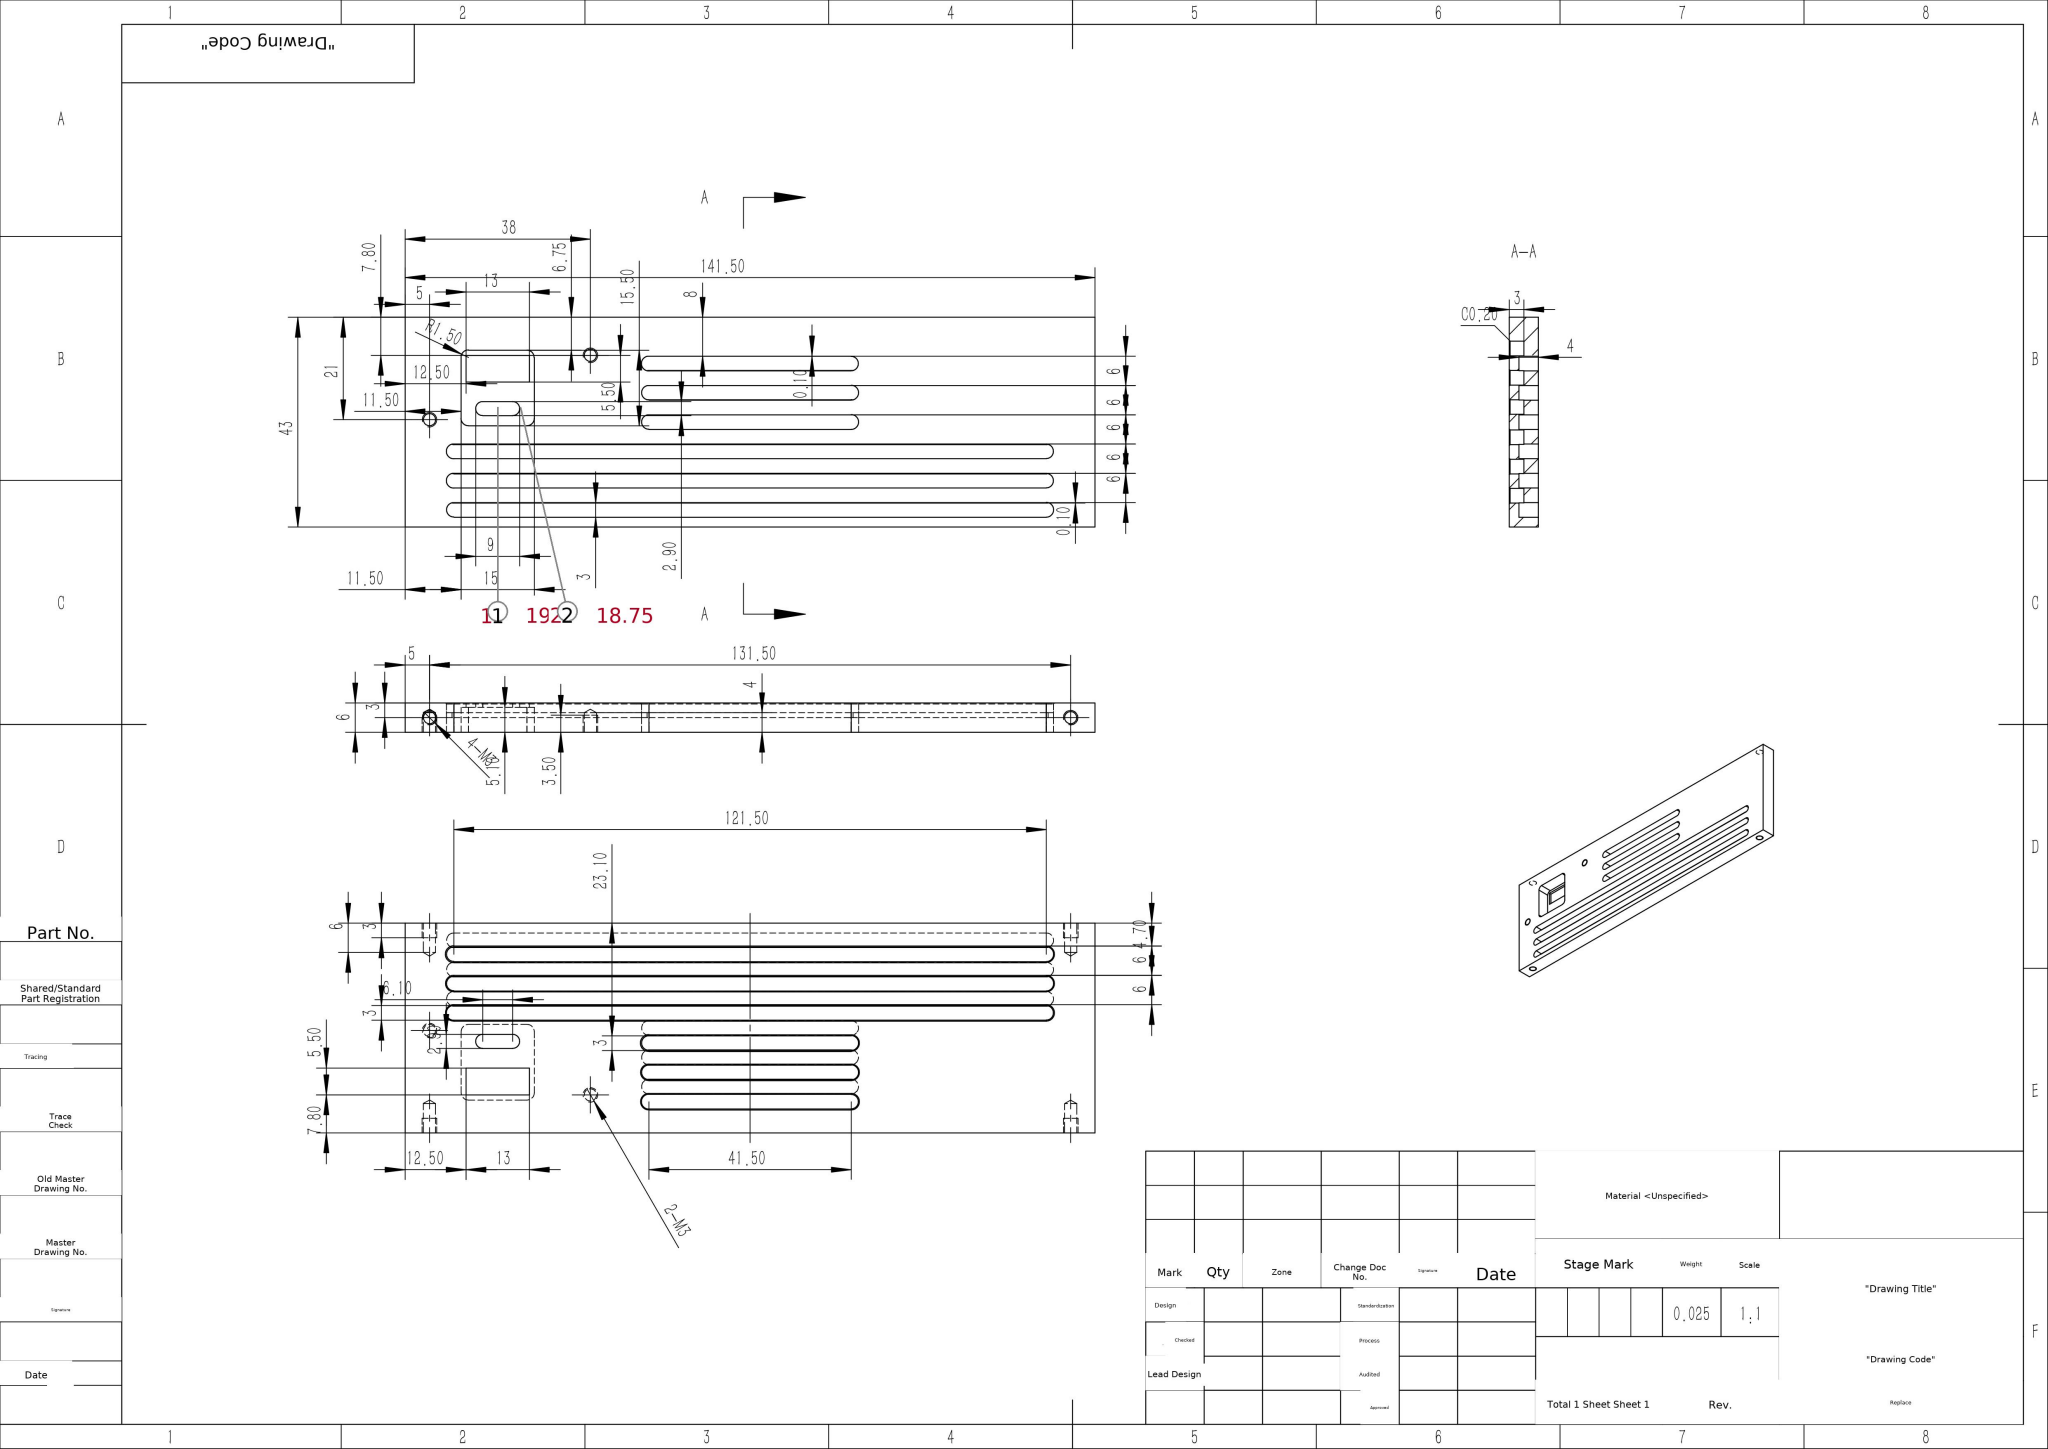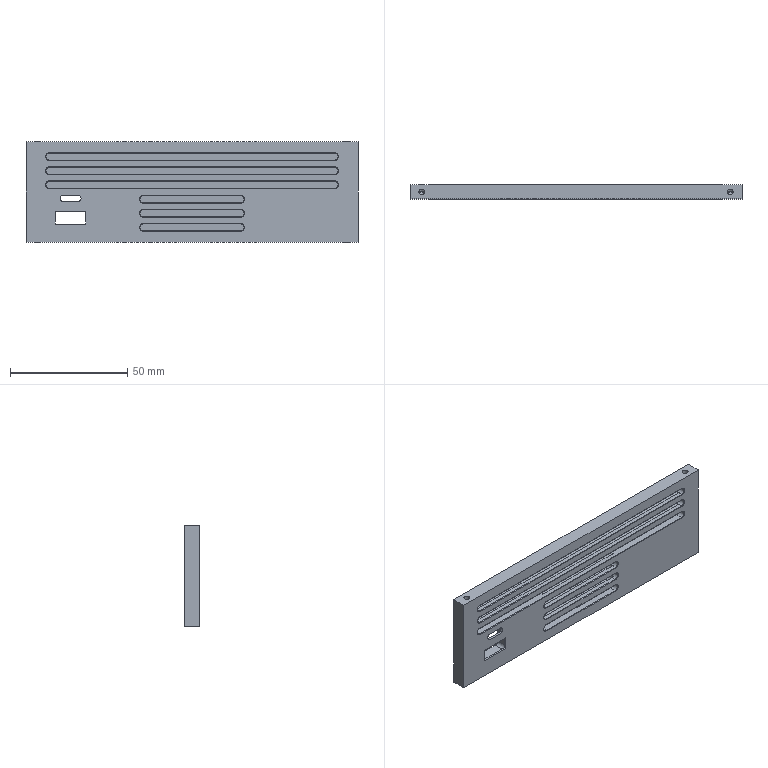Part | SolidWorks | mm | 1 solid | 131 faces | box 141.5 x 6 x 43 mm | volume 24539 mm3 | plane 65 | cylinder 42 | cone 24 | commonest cylinder face diameters 3 x28 2.5 x12 2.9 x2
build123d program:
from build123d import *

# Parameters (mm, degrees)
SKETCH1_W             = 141.5
SKETCH1_H             = 43
BOSS_EXTRUDE1_DEPTH   = 6
CUT_EXTRUDE1_DEPTH    = 4
LPATTERN1_COUNT       = 3
LPATTERN1_PITCH       = 6
CUT_EXTRUDE4_DEPTH    = 3
LPATTERN2_COUNT       = 3
LPATTERN2_PITCH       = 6
CUT_EXTRUDE5_DEPTH    = 4
LPATTERN3_COUNT       = 3
LPATTERN3_PITCH       = 6
CUT_EXTRUDE6_DEPTH    = 3
LPATTERN4_COUNT       = 3
LPATTERN4_PITCH       = 6
SKETCH13_W            = 15
SKETCH13_H            = 15.5
CUT_EXTRUDE7_DEPTH    = 5.1
FILLET1_R             = 1.5
CHAMFER2_SIZE         = 0.2
SKETCH15_W            = 13
SKETCH15_H            = 5.5
CUT_EXTRUDE8_DEPTH    = 5.1
CUT_EXTRUDE9_DEPTH    = 5.1
M3_TAPPED_HOLE3_D     = 2.5
M3_TAPPED_HOLE3_DEPTH = 4
M3_TAPPED_HOLE3_TIP   = 0.7511
M3_TAPPED_HOLE4_D     = 2.5
M3_TAPPED_HOLE4_DEPTH = 4
M3_TAPPED_HOLE4_TIP   = 0.7511


with BuildPart() as part:
    # Sketch1 → Boss-Extrude1 (new body)
    with BuildSketch(Plane(origin=(0, 0, 0), x_dir=(1, 0, 0), z_dir=(0, 1, 0))):
        Rectangle(SKETCH1_W, SKETCH1_H)
    extrude(amount=BOSS_EXTRUDE1_DEPTH)

    # Sketch5 → M3 Tapped Hole1 (revolve, cut)
    with BuildSketch(Plane(origin=(-65.75, 3, -21.5), x_dir=(0, 1, 0), z_dir=(1, 0, 0))):
        Polygon((0, 0), (0, 6.751), (1.25, 6), (1.25, 0), align=None)
    m3_tapped_hole1 = revolve(axis=Axis((-65.75, 3, -27.85), (0, 0, 1)), mode=Mode.SUBTRACT)

    # Sketch7 → M3 Tapped Hole2 (revolve, cut)
    with BuildSketch(Plane(origin=(-65.75, 3, 21.5), x_dir=(0, -1, 0), z_dir=(1, 0, 0))):
        Polygon((0, 0), (0, 6.751), (1.25, 6), (1.25, 0), align=None)
    m3_tapped_hole2 = revolve(axis=Axis((-65.75, 3, 27.85), (0, 0, -1)), mode=Mode.SUBTRACT)

    # Sketch9 → Cut-Extrude1 (cut)
    with BuildSketch(Plane(origin=(0, 6, 0), x_dir=(1, 0, 0), z_dir=(0, 1, 0))):
        with BuildLine():
            Line((60.75, -19.5), (-60.75, -19.5))
            ThreePointArc((-60.75, -19.5), (-62.25, -18), (-60.75, -16.5))
            Line((-60.75, -16.5), (60.75, -16.5))
            ThreePointArc((60.75, -16.5), (62.25, -18), (60.75, -19.5))
        make_face()
    cut_extrude1 = extrude(amount=-CUT_EXTRUDE1_DEPTH, mode=Mode.SUBTRACT)

    # LPattern1: Cut-Extrude1 ×3
    with Locations(*[(0, 0, -i * LPATTERN1_PITCH) for i in range(1, LPATTERN1_COUNT)]):
        add(cut_extrude1, mode=Mode.SUBTRACT)

    # Sketch10 → Cut-Extrude4 (cut)
    with BuildSketch(Plane.XZ):
        with BuildLine():
            Line((-60.75, 16.6), (60.75, 16.6))
            ThreePointArc((60.75, 16.6), (62.25, 15.1), (60.75, 13.6))
            Line((60.75, 13.6), (-60.75, 13.6))
            ThreePointArc((-60.75, 13.6), (-62.25, 15.1), (-60.75, 16.6))
        make_face()
    cut_extrude4 = extrude(amount=-CUT_EXTRUDE4_DEPTH, mode=Mode.SUBTRACT)

    # LPattern2: Cut-Extrude4 ×3
    with Locations(*[(0, 0, -i * LPATTERN2_PITCH) for i in range(1, LPATTERN2_COUNT)]):
        add(cut_extrude4, mode=Mode.SUBTRACT)

    # Sketch11 → Cut-Extrude5 (cut)
    with BuildSketch(Plane(origin=(0, 6, 0), x_dir=(1, 0, 0), z_dir=(0, 1, 0))):
        with BuildLine():
            Line((20.75, -1.5), (-20.75, -1.5))
            ThreePointArc((-20.75, -1.5), (-22.25, 0), (-20.75, 1.5))
            Line((-20.75, 1.5), (20.75, 1.5))
            ThreePointArc((20.75, 1.5), (22.25, 0), (20.75, -1.5))
        make_face()
    cut_extrude5 = extrude(amount=-CUT_EXTRUDE5_DEPTH, mode=Mode.SUBTRACT)

    # LPattern3: Cut-Extrude5 ×3
    with Locations(*[(0, 0, -i * LPATTERN3_PITCH) for i in range(1, LPATTERN3_COUNT)]):
        add(cut_extrude5, mode=Mode.SUBTRACT)

    # Sketch12 → Cut-Extrude6 (cut)
    with BuildSketch(Plane.XZ):
        with BuildLine():
            Line((-20.75, -1.6), (20.75, -1.6))
            ThreePointArc((20.75, -1.6), (22.25, -3.1), (20.75, -4.6))
            Line((20.75, -4.6), (-20.75, -4.6))
            ThreePointArc((-20.75, -4.6), (-22.25, -3.1), (-20.75, -1.6))
        make_face()
    cut_extrude6 = extrude(amount=-CUT_EXTRUDE6_DEPTH, mode=Mode.SUBTRACT)

    # LPattern4: Cut-Extrude6 ×3
    with Locations(*[(0, 0, -i * LPATTERN4_PITCH) for i in range(1, LPATTERN4_COUNT)]):
        add(cut_extrude6, mode=Mode.SUBTRACT)

    # Sketch13 → Cut-Extrude7 (cut)
    with BuildSketch(Plane.XZ.offset(-6)):
        with Locations((-51.75, -7)):
            Rectangle(SKETCH13_W, SKETCH13_H)
    extrude(amount=CUT_EXTRUDE7_DEPTH, mode=Mode.SUBTRACT)

    # Fillet1
    fillet1_edges = [part.edges().sort_by_distance(p)[0] for p in [
        (-44.25, 3.45, -14.75),
        (-44.25, 3.45, 0.75),
        (-59.25, 3.45, 0.75),
        (-59.25, 3.45, -14.75),
    ]]
    fillet(fillet1_edges, radius=FILLET1_R)

    # Chamfer2
    chamfer2_edges = [part.edges().sort_by_distance(p)[0] for p in [
        (0, 0, 7.6),
        (62.25, 0, 9.1),
        (-62.25, 0, 9.1),
        (0, 0, 4.6),
        (0, 0, 1.6),
        (62.25, 0, 3.1),
        (-62.25, 0, 3.1),
        (-22.25, 0, -3.1),
        (0, 0, -4.6),
        (22.25, 0, -3.1),
        (0, 0, -1.6),
        (-22.25, 0, -9.1),
        (0, 0, -10.6),
        (22.25, 0, -9.1),
        (0, 0, -7.6),
        (-22.25, 0, -15.1),
        (0, 0, -16.6),
        (22.25, 0, -15.1),
        (0, 0, -13.6),
        (0, 0, 16.6),
        (0, 0, 13.6),
        (62.25, 0, 15.1),
        (-62.25, 0, 15.1),
        (0, 0, 10.6),
    ]]
    chamfer(chamfer2_edges, length=CHAMFER2_SIZE)

    # Sketch15 → Cut-Extrude8 (cut)
    with BuildSketch(Plane(origin=(0, 0.9, 0), x_dir=(1, 0, 0), z_dir=(0, 1, 0))):
        with Locations((-51.75, 10.95)):
            Rectangle(SKETCH15_W, SKETCH15_H)
    extrude(amount=-CUT_EXTRUDE8_DEPTH, mode=Mode.SUBTRACT)

    # Sketch16 → Cut-Extrude9 (cut)
    with BuildSketch(Plane(origin=(0, 0.9, 0), x_dir=(1, 0, 0), z_dir=(0, 1, 0))):
        with BuildLine():
            Line((-54.8, 4.2), (-48.7, 4.2))
            ThreePointArc((-48.7, 4.2), (-47.25, 2.75), (-48.7, 1.3))
            Line((-48.7, 1.3), (-54.8, 1.3))
            ThreePointArc((-54.8, 1.3), (-56.25, 2.75), (-54.8, 4.2))
        make_face()
    extrude(amount=-CUT_EXTRUDE9_DEPTH, mode=Mode.SUBTRACT)

    # M3 Tapped Hole3
    with Locations(Plane(origin=(0, 6, 0), x_dir=(-1, 0, 0), z_dir=(0, 1, 0))):
        with Locations((32.75, -13.7)):
            Hole(M3_TAPPED_HOLE3_D / 2, depth=M3_TAPPED_HOLE3_DEPTH)
            with Locations((0, 0, -(M3_TAPPED_HOLE3_DEPTH + M3_TAPPED_HOLE3_TIP / 2))):  # 118° drill point
                Cone(0, M3_TAPPED_HOLE3_D / 2, M3_TAPPED_HOLE3_TIP, mode=Mode.SUBTRACT)

    # M3 Tapped Hole4
    with Locations(Plane(origin=(0, 6, 0), x_dir=(-1, 0, 0), z_dir=(0, 1, 0))):
        with Locations((65.75, -0.5)):
            Hole(M3_TAPPED_HOLE4_D / 2, depth=M3_TAPPED_HOLE4_DEPTH)
            with Locations((0, 0, -(M3_TAPPED_HOLE4_DEPTH + M3_TAPPED_HOLE4_TIP / 2))):  # 118° drill point
                Cone(0, M3_TAPPED_HOLE4_D / 2, M3_TAPPED_HOLE4_TIP, mode=Mode.SUBTRACT)

    # Mirror1: M3 Tapped Hole1, M3 Tapped Hole2 across plane
    add(m3_tapped_hole1.mirror(Plane(origin=(0, 0, 0), x_dir=(0, 0, 1), z_dir=(1, 0, 0))), mode=Mode.SUBTRACT)
    add(m3_tapped_hole2.mirror(Plane(origin=(0, 0, 0), x_dir=(0, 0, 1), z_dir=(1, 0, 0))), mode=Mode.SUBTRACT)


solid = part.part